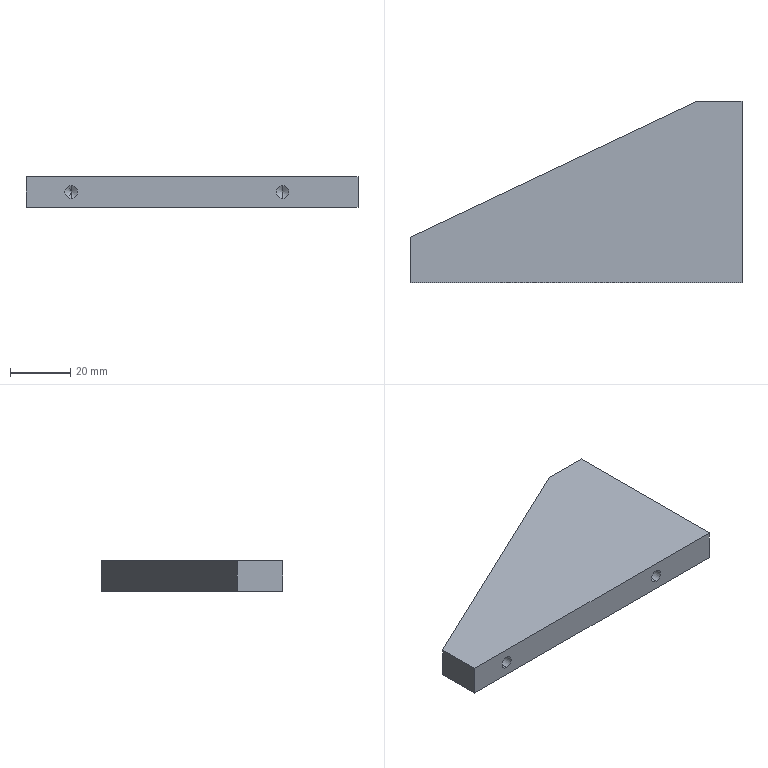Component | SolidWorks | SL021-102-4067.SL4PRT-1 | 1 solid | 23 faces | box 110 x 60 x 10 mm | volume 43715 mm3 | cylinder 8 | cone 8 | plane 7 | commonest cylinder face diameters 4.2 x8 | material AL6061
build123d program:
from build123d import *

# Parameters (mm, degrees)
BOSS_EXTRUDE1_DEPTH   = 5
M5_TAPPED_HOLE1_D     = 4.2
M5_TAPPED_HOLE1_DEPTH = 16
M5_TAPPED_HOLE1_TIP   = 1.262
M5_TAPPED_HOLE2_D     = 4.2
M5_TAPPED_HOLE2_DEPTH = 16
M5_TAPPED_HOLE2_TIP   = 1.262


with BuildPart() as part:
    # Sketch1 → Boss-Extrude1 (new, symmetric)
    with BuildSketch(Plane.XY):
        Polygon((0, 0), (0, 60), (15, 60), (110, 15), (110, 0), align=None)
    extrude(amount=BOSS_EXTRUDE1_DEPTH, both=True)

    # M5 Tapped Hole1
    with Locations(Plane.ZY):
        with Locations((0, 50), (0, 15)):
            Hole(M5_TAPPED_HOLE1_D / 2, depth=M5_TAPPED_HOLE1_DEPTH)
            with Locations((0, 0, -(M5_TAPPED_HOLE1_DEPTH + M5_TAPPED_HOLE1_TIP / 2))):  # 118° drill point
                Cone(0, M5_TAPPED_HOLE1_D / 2, M5_TAPPED_HOLE1_TIP, mode=Mode.SUBTRACT)

    # M5 Tapped Hole2
    with Locations(Plane(origin=(0, 0, 0), x_dir=(-1, 0, 0), z_dir=(0, -1, 0))):
        with Locations((-25, 0), (-95, 0)):
            Hole(M5_TAPPED_HOLE2_D / 2, depth=M5_TAPPED_HOLE2_DEPTH)
            with Locations((0, 0, -(M5_TAPPED_HOLE2_DEPTH + M5_TAPPED_HOLE2_TIP / 2))):  # 118° drill point
                Cone(0, M5_TAPPED_HOLE2_D / 2, M5_TAPPED_HOLE2_TIP, mode=Mode.SUBTRACT)


solid = part.part

# Placed as in the assembly
solid = solid.moved(Location((13.837, -10.499, -86.378), (-180, 0, 180)))
STEP:
#1=COLOUR_RGB('',0.7922,0.8196,0.9333);
#2=FILL_AREA_STYLE_COLOUR('',#1);
#3=FILL_AREA_STYLE('',(#2));
#4=SURFACE_STYLE_FILL_AREA(#3);
#5=SURFACE_SIDE_STYLE('',(#4));
#6=SURFACE_STYLE_USAGE(.BOTH.,#5);
#7=PRESENTATION_STYLE_ASSIGNMENT((#6));
#8=CARTESIAN_POINT('',(-0.4395,0.2166,-3.483));
#9=VERTEX_POINT('',#8);
#10=CARTESIAN_POINT('',(-0.4395,0.2166,-3.318));
#11=VERTEX_POINT('',#10);
#12=CARTESIAN_POINT('',(-0.4395,0.2166,-3.401));
#13=DIRECTION('',(-0.,-1.,0.));
#14=DIRECTION('',(0.,0.,1.));
#15=AXIS2_PLACEMENT_3D('',#12,#13,#14);
#16=CIRCLE('',#15,0.08268);
#17=EDGE_CURVE('',#9,#11,#16,.T.);
#18=ORIENTED_EDGE('',*,*,#17,.F.);
#19=CARTESIAN_POINT('',(-0.4395,-0.4133,-3.483));
#20=VERTEX_POINT('',#19);
#21=CARTESIAN_POINT('',(-0.4395,-0.4133,-3.483));
#22=DIRECTION('',(-0.,-1.,0.));
#23=VECTOR('',#22,39.37);
#24=LINE('',#21,#23);
#25=EDGE_CURVE('',#9,#20,#24,.T.);
#26=ORIENTED_EDGE('',*,*,#25,.T.);
#27=CARTESIAN_POINT('',(-0.4395,-0.4133,-3.318));
#28=VERTEX_POINT('',#27);
#29=CARTESIAN_POINT('',(-0.4395,-0.4133,-3.401));
#30=DIRECTION('',(-0.,-1.,0.));
#31=DIRECTION('',(0.,0.,1.));
#32=AXIS2_PLACEMENT_3D('',#29,#30,#31);
#33=CIRCLE('',#32,0.08268);
#34=EDGE_CURVE('',#20,#28,#33,.T.);
#35=ORIENTED_EDGE('',*,*,#34,.T.);
#36=CARTESIAN_POINT('',(-0.4395,-0.4133,-3.318));
#37=DIRECTION('',(-0.,-1.,0.));
#38=VECTOR('',#37,39.37);
#39=LINE('',#36,#38);
#40=EDGE_CURVE('',#11,#28,#39,.T.);
#41=ORIENTED_EDGE('',*,*,#40,.F.);
#42=EDGE_LOOP('',(#18,#26,#35,#41));
#43=FACE_OUTER_BOUND('',#42,.T.);
#44=CARTESIAN_POINT('',(-0.4395,-0.4133,-3.401));
#45=DIRECTION('',(-0.,-1.,0.));
#46=DIRECTION('',(0.,0.,1.));
#47=AXIS2_PLACEMENT_3D('',#44,#45,#46);
#48=CYLINDRICAL_SURFACE('',#47,0.08268);
#49=ADVANCED_FACE('',(#43),#48,.F.);
#50=CARTESIAN_POINT('',(-0.4395,0.2663,-3.401));
#51=VERTEX_POINT('',#50);
#52=CARTESIAN_POINT('',(-0.4395,0.2166,-3.318));
#53=DIRECTION('',(0.,-0.515,0.8572));
#54=VECTOR('',#53,39.37);
#55=LINE('',#52,#54);
#56=EDGE_CURVE('',#51,#11,#55,.T.);
#57=ORIENTED_EDGE('',*,*,#56,.F.);
#58=CARTESIAN_POINT('',(-0.4395,0.2166,-3.483));
#59=DIRECTION('',(-0.,-0.515,-0.8572));
#60=VECTOR('',#59,39.37);
#61=LINE('',#58,#60);
#62=EDGE_CURVE('',#51,#9,#61,.T.);
#63=ORIENTED_EDGE('',*,*,#62,.T.);
#64=ORIENTED_EDGE('',*,*,#17,.T.);
#65=EDGE_LOOP('',(#57,#63,#64));
#66=FACE_OUTER_BOUND('',#65,.T.);
#67=CARTESIAN_POINT('',(-0.4395,0.2166,-3.401));
#68=DIRECTION('',(-0.,-1.,0.));
#69=DIRECTION('',(0.,0.,1.));
#70=AXIS2_PLACEMENT_3D('',#67,#68,#69);
#71=CONICAL_SURFACE('',#70,0.08268,1.03);
#72=ADVANCED_FACE('',(#66),#71,.F.);
#73=CARTESIAN_POINT('',(-3.195,0.2166,-3.483));
#74=VERTEX_POINT('',#73);
#75=CARTESIAN_POINT('',(-3.195,0.2166,-3.318));
#76=VERTEX_POINT('',#75);
#77=CARTESIAN_POINT('',(-3.195,0.2166,-3.401));
#78=DIRECTION('',(-0.,-1.,0.));
#79=DIRECTION('',(0.,0.,1.));
#80=AXIS2_PLACEMENT_3D('',#77,#78,#79);
#81=CIRCLE('',#80,0.08268);
#82=EDGE_CURVE('',#74,#76,#81,.T.);
#83=ORIENTED_EDGE('',*,*,#82,.F.);
#84=CARTESIAN_POINT('',(-3.195,-0.4133,-3.483));
#85=VERTEX_POINT('',#84);
#86=CARTESIAN_POINT('',(-3.195,-0.4133,-3.483));
#87=DIRECTION('',(-0.,-1.,0.));
#88=VECTOR('',#87,39.37);
#89=LINE('',#86,#88);
#90=EDGE_CURVE('',#74,#85,#89,.T.);
#91=ORIENTED_EDGE('',*,*,#90,.T.);
#92=CARTESIAN_POINT('',(-3.195,-0.4133,-3.318));
#93=VERTEX_POINT('',#92);
#94=CARTESIAN_POINT('',(-3.195,-0.4133,-3.401));
#95=DIRECTION('',(-0.,-1.,0.));
#96=DIRECTION('',(0.,0.,1.));
#97=AXIS2_PLACEMENT_3D('',#94,#95,#96);
#98=CIRCLE('',#97,0.08268);
#99=EDGE_CURVE('',#85,#93,#98,.T.);
#100=ORIENTED_EDGE('',*,*,#99,.T.);
#101=CARTESIAN_POINT('',(-3.195,-0.4133,-3.318));
#102=DIRECTION('',(-0.,-1.,0.));
#103=VECTOR('',#102,39.37);
#104=LINE('',#101,#103);
#105=EDGE_CURVE('',#76,#93,#104,.T.);
#106=ORIENTED_EDGE('',*,*,#105,.F.);
#107=EDGE_LOOP('',(#83,#91,#100,#106));
#108=FACE_OUTER_BOUND('',#107,.T.);
#109=CARTESIAN_POINT('',(-3.195,-0.4133,-3.401));
#110=DIRECTION('',(-0.,-1.,0.));
#111=DIRECTION('',(0.,0.,1.));
#112=AXIS2_PLACEMENT_3D('',#109,#110,#111);
#113=CYLINDRICAL_SURFACE('',#112,0.08268);
#114=ADVANCED_FACE('',(#108),#113,.F.);
#115=CARTESIAN_POINT('',(-3.195,0.2663,-3.401));
#116=VERTEX_POINT('',#115);
#117=CARTESIAN_POINT('',(-3.195,0.2166,-3.318));
#118=DIRECTION('',(0.,-0.515,0.8572));
#119=VECTOR('',#118,39.37);
#120=LINE('',#117,#119);
#121=EDGE_CURVE('',#116,#76,#120,.T.);
#122=ORIENTED_EDGE('',*,*,#121,.F.);
#123=CARTESIAN_POINT('',(-3.195,0.2166,-3.483));
#124=DIRECTION('',(-0.,-0.515,-0.8572));
#125=VECTOR('',#124,39.37);
#126=LINE('',#123,#125);
#127=EDGE_CURVE('',#116,#74,#126,.T.);
#128=ORIENTED_EDGE('',*,*,#127,.T.);
#129=ORIENTED_EDGE('',*,*,#82,.T.);
#130=EDGE_LOOP('',(#122,#128,#129));
#131=FACE_OUTER_BOUND('',#130,.T.);
#132=CARTESIAN_POINT('',(-3.195,0.2166,-3.401));
#133=DIRECTION('',(-0.,-1.,0.));
#134=DIRECTION('',(0.,0.,1.));
#135=AXIS2_PLACEMENT_3D('',#132,#133,#134);
#136=CONICAL_SURFACE('',#135,0.08268,1.03);
#137=ADVANCED_FACE('',(#131),#136,.F.);
#138=CARTESIAN_POINT('',(-0.08518,1.555,-3.318));
#139=VERTEX_POINT('',#138);
#140=CARTESIAN_POINT('',(-0.08518,1.555,-3.483));
#141=VERTEX_POINT('',#140);
#142=CARTESIAN_POINT('',(-0.08518,1.555,-3.401));
#143=DIRECTION('',(1.,-0.,0.));
#144=DIRECTION('',(-0.,0.,-1.));
#145=AXIS2_PLACEMENT_3D('',#142,#143,#144);
#146=CIRCLE('',#145,0.08268);
#147=EDGE_CURVE('',#139,#141,#146,.T.);
#148=ORIENTED_EDGE('',*,*,#147,.F.);
#149=CARTESIAN_POINT('',(0.5447,1.555,-3.318));
#150=VERTEX_POINT('',#149);
#151=CARTESIAN_POINT('',(0.5447,1.555,-3.318));
#152=DIRECTION('',(1.,-0.,0.));
#153=VECTOR('',#152,39.37);
#154=LINE('',#151,#153);
#155=EDGE_CURVE('',#139,#150,#154,.T.);
#156=ORIENTED_EDGE('',*,*,#155,.T.);
#157=CARTESIAN_POINT('',(0.5447,1.555,-3.483));
#158=VERTEX_POINT('',#157);
#159=CARTESIAN_POINT('',(0.5447,1.555,-3.401));
#160=DIRECTION('',(1.,-0.,0.));
#161=DIRECTION('',(0.,0.,-1.));
#162=AXIS2_PLACEMENT_3D('',#159,#160,#161);
#163=CIRCLE('',#162,0.08268);
#164=EDGE_CURVE('',#150,#158,#163,.T.);
#165=ORIENTED_EDGE('',*,*,#164,.T.);
#166=CARTESIAN_POINT('',(0.5447,1.555,-3.483));
#167=DIRECTION('',(1.,-0.,0.));
#168=VECTOR('',#167,39.37);
#169=LINE('',#166,#168);
#170=EDGE_CURVE('',#141,#158,#169,.T.);
#171=ORIENTED_EDGE('',*,*,#170,.F.);
#172=EDGE_LOOP('',(#148,#156,#165,#171));
#173=FACE_OUTER_BOUND('',#172,.T.);
#174=CARTESIAN_POINT('',(0.5447,1.555,-3.401));
#175=DIRECTION('',(1.,-0.,0.));
#176=DIRECTION('',(0.,0.,-1.));
#177=AXIS2_PLACEMENT_3D('',#174,#175,#176);
#178=CYLINDRICAL_SURFACE('',#177,0.08268);
#179=ADVANCED_FACE('',(#173),#178,.F.);
#180=CARTESIAN_POINT('',(-0.1349,1.555,-3.401));
#181=VERTEX_POINT('',#180);
#182=CARTESIAN_POINT('',(-0.08518,1.555,-3.483));
#183=DIRECTION('',(0.515,-0.,-0.8572));
#184=VECTOR('',#183,39.37);
#185=LINE('',#182,#184);
#186=EDGE_CURVE('',#181,#141,#185,.T.);
#187=ORIENTED_EDGE('',*,*,#186,.F.);
#188=CARTESIAN_POINT('',(-0.08518,1.555,-3.318));
#189=DIRECTION('',(0.515,0.,0.8572));
#190=VECTOR('',#189,39.37);
#191=LINE('',#188,#190);
#192=EDGE_CURVE('',#181,#139,#191,.T.);
#193=ORIENTED_EDGE('',*,*,#192,.T.);
#194=ORIENTED_EDGE('',*,*,#147,.T.);
#195=EDGE_LOOP('',(#187,#193,#194));
#196=FACE_OUTER_BOUND('',#195,.T.);
#197=CARTESIAN_POINT('',(-0.08518,1.555,-3.401));
#198=DIRECTION('',(1.,-0.,0.));
#199=DIRECTION('',(-0.,0.,-1.));
#200=AXIS2_PLACEMENT_3D('',#197,#198,#199);
#201=CONICAL_SURFACE('',#200,0.08268,1.03);
#202=ADVANCED_FACE('',(#196),#201,.F.);
#203=CARTESIAN_POINT('',(-0.08518,0.1772,-3.318));
#204=VERTEX_POINT('',#203);
#205=CARTESIAN_POINT('',(-0.08518,0.1772,-3.483));
#206=VERTEX_POINT('',#205);
#207=CARTESIAN_POINT('',(-0.08518,0.1772,-3.401));
#208=DIRECTION('',(1.,-0.,0.));
#209=DIRECTION('',(-0.,0.,-1.));
#210=AXIS2_PLACEMENT_3D('',#207,#208,#209);
#211=CIRCLE('',#210,0.08268);
#212=EDGE_CURVE('',#204,#206,#211,.T.);
#213=ORIENTED_EDGE('',*,*,#212,.F.);
#214=CARTESIAN_POINT('',(0.5447,0.1772,-3.318));
#215=VERTEX_POINT('',#214);
#216=CARTESIAN_POINT('',(0.5447,0.1772,-3.318));
#217=DIRECTION('',(1.,-0.,0.));
#218=VECTOR('',#217,39.37);
#219=LINE('',#216,#218);
#220=EDGE_CURVE('',#204,#215,#219,.T.);
#221=ORIENTED_EDGE('',*,*,#220,.T.);
#222=CARTESIAN_POINT('',(0.5447,0.1772,-3.483));
#223=VERTEX_POINT('',#222);
#224=CARTESIAN_POINT('',(0.5447,0.1772,-3.401));
#225=DIRECTION('',(1.,-0.,0.));
#226=DIRECTION('',(0.,0.,-1.));
#227=AXIS2_PLACEMENT_3D('',#224,#225,#226);
#228=CIRCLE('',#227,0.08268);
#229=EDGE_CURVE('',#215,#223,#228,.T.);
#230=ORIENTED_EDGE('',*,*,#229,.T.);
#231=CARTESIAN_POINT('',(0.5447,0.1772,-3.483));
#232=DIRECTION('',(1.,-0.,0.));
#233=VECTOR('',#232,39.37);
#234=LINE('',#231,#233);
#235=EDGE_CURVE('',#206,#223,#234,.T.);
#236=ORIENTED_EDGE('',*,*,#235,.F.);
#237=EDGE_LOOP('',(#213,#221,#230,#236));
#238=FACE_OUTER_BOUND('',#237,.T.);
#239=CARTESIAN_POINT('',(0.5447,0.1772,-3.401));
#240=DIRECTION('',(1.,-0.,0.));
#241=DIRECTION('',(0.,0.,-1.));
#242=AXIS2_PLACEMENT_3D('',#239,#240,#241);
#243=CYLINDRICAL_SURFACE('',#242,0.08268);
#244=ADVANCED_FACE('',(#238),#243,.F.);
#245=CARTESIAN_POINT('',(-0.1349,0.1772,-3.401));
#246=VERTEX_POINT('',#245);
#247=CARTESIAN_POINT('',(-0.08518,0.1772,-3.483));
#248=DIRECTION('',(0.515,-0.,-0.8572));
#249=VECTOR('',#248,39.37);
#250=LINE('',#247,#249);
#251=EDGE_CURVE('',#246,#206,#250,.T.);
#252=ORIENTED_EDGE('',*,*,#251,.F.);
#253=CARTESIAN_POINT('',(-0.08518,0.1772,-3.318));
#254=DIRECTION('',(0.515,0.,0.8572));
#255=VECTOR('',#254,39.37);
#256=LINE('',#253,#255);
#257=EDGE_CURVE('',#246,#204,#256,.T.);
#258=ORIENTED_EDGE('',*,*,#257,.T.);
#259=ORIENTED_EDGE('',*,*,#212,.T.);
#260=EDGE_LOOP('',(#252,#258,#259));
#261=FACE_OUTER_BOUND('',#260,.T.);
#262=CARTESIAN_POINT('',(-0.08518,0.1772,-3.401));
#263=DIRECTION('',(1.,-0.,0.));
#264=DIRECTION('',(-0.,0.,-1.));
#265=AXIS2_PLACEMENT_3D('',#262,#263,#264);
#266=CONICAL_SURFACE('',#265,0.08268,1.03);
#267=ADVANCED_FACE('',(#261),#266,.F.);
#268=CARTESIAN_POINT('',(-0.4395,-0.4133,-3.401));
#269=DIRECTION('',(-0.,-1.,0.));
#270=DIRECTION('',(0.,0.,1.));
#271=AXIS2_PLACEMENT_3D('',#268,#269,#270);
#272=CIRCLE('',#271,0.08268);
#273=EDGE_CURVE('',#28,#20,#272,.T.);
#274=ORIENTED_EDGE('',*,*,#273,.F.);
#275=ORIENTED_EDGE('',*,*,#34,.F.);
#276=EDGE_LOOP('',(#274,#275));
#277=FACE_BOUND('',#276,.T.);
#278=CARTESIAN_POINT('',(-3.195,-0.4133,-3.401));
#279=DIRECTION('',(-0.,-1.,0.));
#280=DIRECTION('',(0.,0.,1.));
#281=AXIS2_PLACEMENT_3D('',#278,#279,#280);
#282=CIRCLE('',#281,0.08268);
#283=EDGE_CURVE('',#93,#85,#282,.T.);
#284=ORIENTED_EDGE('',*,*,#283,.F.);
#285=ORIENTED_EDGE('',*,*,#99,.F.);
#286=EDGE_LOOP('',(#284,#285));
#287=FACE_BOUND('',#286,.T.);
#288=CARTESIAN_POINT('',(0.5447,-0.4133,-3.204));
#289=VERTEX_POINT('',#288);
#290=CARTESIAN_POINT('',(-3.786,-0.4133,-3.204));
#291=VERTEX_POINT('',#290);
#292=CARTESIAN_POINT('',(-3.786,-0.4133,-3.204));
#293=DIRECTION('',(-1.,0.,-0.));
#294=VECTOR('',#293,39.37);
#295=LINE('',#292,#294);
#296=EDGE_CURVE('',#289,#291,#295,.T.);
#297=ORIENTED_EDGE('',*,*,#296,.T.);
#298=CARTESIAN_POINT('',(-3.786,-0.4133,-3.598));
#299=VERTEX_POINT('',#298);
#300=CARTESIAN_POINT('',(-3.786,-0.4133,-3.598));
#301=DIRECTION('',(0.,0.,1.));
#302=VECTOR('',#301,39.37);
#303=LINE('',#300,#302);
#304=EDGE_CURVE('',#299,#291,#303,.T.);
#305=ORIENTED_EDGE('',*,*,#304,.F.);
#306=CARTESIAN_POINT('',(0.5447,-0.4133,-3.598));
#307=VERTEX_POINT('',#306);
#308=CARTESIAN_POINT('',(-3.786,-0.4133,-3.598));
#309=DIRECTION('',(-1.,0.,-0.));
#310=VECTOR('',#309,39.37);
#311=LINE('',#308,#310);
#312=EDGE_CURVE('',#307,#299,#311,.T.);
#313=ORIENTED_EDGE('',*,*,#312,.F.);
#314=CARTESIAN_POINT('',(0.5447,-0.4133,-3.598));
#315=DIRECTION('',(0.,0.,1.));
#316=VECTOR('',#315,39.37);
#317=LINE('',#314,#316);
#318=EDGE_CURVE('',#307,#289,#317,.T.);
#319=ORIENTED_EDGE('',*,*,#318,.T.);
#320=EDGE_LOOP('',(#297,#305,#313,#319));
#321=FACE_OUTER_BOUND('',#320,.T.);
#322=CARTESIAN_POINT('',(-3.786,-0.4133,-3.598));
#323=DIRECTION('',(0.,1.,-0.));
#324=DIRECTION('',(1.,-0.,0.));
#325=AXIS2_PLACEMENT_3D('',#322,#323,#324);
#326=PLANE('',#325);
#327=ADVANCED_FACE('',(#277,#287,#321),#326,.F.);
#328=CARTESIAN_POINT('',(-3.786,0.1772,-3.204));
#329=VERTEX_POINT('',#328);
#330=CARTESIAN_POINT('',(-3.786,0.1772,-3.204));
#331=DIRECTION('',(0.,1.,-0.));
#332=VECTOR('',#331,39.37);
#333=LINE('',#330,#332);
#334=EDGE_CURVE('',#291,#329,#333,.T.);
#335=ORIENTED_EDGE('',*,*,#334,.T.);
#336=CARTESIAN_POINT('',(-3.786,0.1772,-3.598));
#337=VERTEX_POINT('',#336);
#338=CARTESIAN_POINT('',(-3.786,0.1772,-3.598));
#339=DIRECTION('',(0.,0.,1.));
#340=VECTOR('',#339,39.37);
#341=LINE('',#338,#340);
#342=EDGE_CURVE('',#337,#329,#341,.T.);
#343=ORIENTED_EDGE('',*,*,#342,.F.);
#344=CARTESIAN_POINT('',(-3.786,0.1772,-3.598));
#345=DIRECTION('',(0.,1.,-0.));
#346=VECTOR('',#345,39.37);
#347=LINE('',#344,#346);
#348=EDGE_CURVE('',#299,#337,#347,.T.);
#349=ORIENTED_EDGE('',*,*,#348,.F.);
#350=ORIENTED_EDGE('',*,*,#304,.T.);
#351=EDGE_LOOP('',(#335,#343,#349,#350));
#352=FACE_OUTER_BOUND('',#351,.T.);
#353=CARTESIAN_POINT('',(-3.786,0.1772,-3.598));
#354=DIRECTION('',(1.,-0.,-0.));
#355=DIRECTION('',(-0.,-0.,-1.));
#356=AXIS2_PLACEMENT_3D('',#353,#354,#355);
#357=PLANE('',#356);
#358=ADVANCED_FACE('',(#352),#357,.F.);
#359=CARTESIAN_POINT('',(-0.04581,1.949,-3.204));
#360=VERTEX_POINT('',#359);
#361=CARTESIAN_POINT('',(-0.04581,1.949,-3.204));
#362=DIRECTION('',(0.9037,0.4281,0.));
#363=VECTOR('',#362,39.37);
#364=LINE('',#361,#363);
#365=EDGE_CURVE('',#329,#360,#364,.T.);
#366=ORIENTED_EDGE('',*,*,#365,.T.);
#367=CARTESIAN_POINT('',(-0.04581,1.949,-3.598));
#368=VERTEX_POINT('',#367);
#369=CARTESIAN_POINT('',(-0.04581,1.949,-3.598));
#370=DIRECTION('',(0.,0.,1.));
#371=VECTOR('',#370,39.37);
#372=LINE('',#369,#371);
#373=EDGE_CURVE('',#368,#360,#372,.T.);
#374=ORIENTED_EDGE('',*,*,#373,.F.);
#375=CARTESIAN_POINT('',(-0.04581,1.949,-3.598));
#376=DIRECTION('',(0.9037,0.4281,0.));
#377=VECTOR('',#376,39.37);
#378=LINE('',#375,#377);
#379=EDGE_CURVE('',#337,#368,#378,.T.);
#380=ORIENTED_EDGE('',*,*,#379,.F.);
#381=ORIENTED_EDGE('',*,*,#342,.T.);
#382=EDGE_LOOP('',(#366,#374,#380,#381));
#383=FACE_OUTER_BOUND('',#382,.T.);
#384=CARTESIAN_POINT('',(-0.04581,1.949,-3.598));
#385=DIRECTION('',(0.4281,-0.9037,0.));
#386=DIRECTION('',(-0.9037,-0.4281,-0.));
#387=AXIS2_PLACEMENT_3D('',#384,#385,#386);
#388=PLANE('',#387);
#389=ADVANCED_FACE('',(#383),#388,.F.);
#390=CARTESIAN_POINT('',(0.5447,1.949,-3.204));
#391=VERTEX_POINT('',#390);
#392=CARTESIAN_POINT('',(0.5447,1.949,-3.204));
#393=DIRECTION('',(1.,-0.,0.));
#394=VECTOR('',#393,39.37);
#395=LINE('',#392,#394);
#396=EDGE_CURVE('',#360,#391,#395,.T.);
#397=ORIENTED_EDGE('',*,*,#396,.T.);
#398=CARTESIAN_POINT('',(0.5447,1.949,-3.598));
#399=VERTEX_POINT('',#398);
#400=CARTESIAN_POINT('',(0.5447,1.949,-3.598));
#401=DIRECTION('',(0.,0.,1.));
#402=VECTOR('',#401,39.37);
#403=LINE('',#400,#402);
#404=EDGE_CURVE('',#399,#391,#403,.T.);
#405=ORIENTED_EDGE('',*,*,#404,.F.);
#406=CARTESIAN_POINT('',(0.5447,1.949,-3.598));
#407=DIRECTION('',(1.,-0.,0.));
#408=VECTOR('',#407,39.37);
#409=LINE('',#406,#408);
#410=EDGE_CURVE('',#368,#399,#409,.T.);
#411=ORIENTED_EDGE('',*,*,#410,.F.);
#412=ORIENTED_EDGE('',*,*,#373,.T.);
#413=EDGE_LOOP('',(#397,#405,#411,#412));
#414=FACE_OUTER_BOUND('',#413,.T.);
#415=CARTESIAN_POINT('',(0.5447,1.949,-3.598));
#416=DIRECTION('',(-0.,-1.,0.));
#417=DIRECTION('',(0.,0.,1.));
#418=AXIS2_PLACEMENT_3D('',#415,#416,#417);
#419=PLANE('',#418);
#420=ADVANCED_FACE('',(#414),#419,.F.);
#421=CARTESIAN_POINT('',(0.5447,1.555,-3.401));
#422=DIRECTION('',(1.,-0.,0.));
#423=DIRECTION('',(0.,0.,-1.));
#424=AXIS2_PLACEMENT_3D('',#421,#422,#423);
#425=CIRCLE('',#424,0.08268);
#426=EDGE_CURVE('',#158,#150,#425,.T.);
#427=ORIENTED_EDGE('',*,*,#426,.F.);
#428=ORIENTED_EDGE('',*,*,#164,.F.);
#429=EDGE_LOOP('',(#427,#428));
#430=FACE_BOUND('',#429,.T.);
#431=CARTESIAN_POINT('',(0.5447,0.1772,-3.401));
#432=DIRECTION('',(1.,-0.,0.));
#433=DIRECTION('',(0.,0.,-1.));
#434=AXIS2_PLACEMENT_3D('',#431,#432,#433);
#435=CIRCLE('',#434,0.08268);
#436=EDGE_CURVE('',#223,#215,#435,.T.);
#437=ORIENTED_EDGE('',*,*,#436,.F.);
#438=ORIENTED_EDGE('',*,*,#229,.F.);
#439=EDGE_LOOP('',(#437,#438));
#440=FACE_BOUND('',#439,.T.);
#441=CARTESIAN_POINT('',(0.5447,-0.4133,-3.204));
#442=DIRECTION('',(-0.,-1.,0.));
#443=VECTOR('',#442,39.37);
#444=LINE('',#441,#443);
#445=EDGE_CURVE('',#391,#289,#444,.T.);
#446=ORIENTED_EDGE('',*,*,#445,.T.);
#447=ORIENTED_EDGE('',*,*,#318,.F.);
#448=CARTESIAN_POINT('',(0.5447,-0.4133,-3.598));
#449=DIRECTION('',(-0.,-1.,0.));
#450=VECTOR('',#449,39.37);
#451=LINE('',#448,#450);
#452=EDGE_CURVE('',#399,#307,#451,.T.);
#453=ORIENTED_EDGE('',*,*,#452,.F.);
#454=ORIENTED_EDGE('',*,*,#404,.T.);
#455=EDGE_LOOP('',(#446,#447,#453,#454));
#456=FACE_OUTER_BOUND('',#455,.T.);
#457=CARTESIAN_POINT('',(0.5447,-0.4133,-3.598));
#458=DIRECTION('',(-1.,0.,0.));
#459=DIRECTION('',(0.,0.,1.));
#460=AXIS2_PLACEMENT_3D('',#457,#458,#459);
#461=PLANE('',#460);
#462=ADVANCED_FACE('',(#430,#440,#456),#461,.F.);
#463=ORIENTED_EDGE('',*,*,#312,.T.);
#464=ORIENTED_EDGE('',*,*,#348,.T.);
#465=ORIENTED_EDGE('',*,*,#379,.T.);
#466=ORIENTED_EDGE('',*,*,#410,.T.);
#467=ORIENTED_EDGE('',*,*,#452,.T.);
#468=EDGE_LOOP('',(#463,#464,#465,#466,#467));
#469=FACE_OUTER_BOUND('',#468,.T.);
#470=CARTESIAN_POINT('',(0.5447,-0.4133,-3.598));
#471=DIRECTION('',(-0.,0.,1.));
#472=DIRECTION('',(1.,-0.,0.));
#473=AXIS2_PLACEMENT_3D('',#470,#471,#472);
#474=PLANE('',#473);
#475=ADVANCED_FACE('',(#469),#474,.F.);
#476=ORIENTED_EDGE('',*,*,#296,.F.);
#477=ORIENTED_EDGE('',*,*,#445,.F.);
#478=ORIENTED_EDGE('',*,*,#396,.F.);
#479=ORIENTED_EDGE('',*,*,#365,.F.);
#480=ORIENTED_EDGE('',*,*,#334,.F.);
#481=EDGE_LOOP('',(#476,#477,#478,#479,#480));
#482=FACE_OUTER_BOUND('',#481,.T.);
#483=CARTESIAN_POINT('',(0.5447,-0.4133,-3.204));
#484=DIRECTION('',(-0.,0.,1.));
#485=DIRECTION('',(1.,-0.,0.));
#486=AXIS2_PLACEMENT_3D('',#483,#484,#485);
#487=PLANE('',#486);
#488=ADVANCED_FACE('',(#482),#487,.T.);
#489=ORIENTED_EDGE('',*,*,#257,.F.);
#490=ORIENTED_EDGE('',*,*,#251,.T.);
#491=CARTESIAN_POINT('',(-0.08518,0.1772,-3.401));
#492=DIRECTION('',(1.,-0.,0.));
#493=DIRECTION('',(-0.,0.,-1.));
#494=AXIS2_PLACEMENT_3D('',#491,#492,#493);
#495=CIRCLE('',#494,0.08268);
#496=EDGE_CURVE('',#206,#204,#495,.T.);
#497=ORIENTED_EDGE('',*,*,#496,.T.);
#498=EDGE_LOOP('',(#489,#490,#497));
#499=FACE_OUTER_BOUND('',#498,.T.);
#500=CARTESIAN_POINT('',(-0.08518,0.1772,-3.401));
#501=DIRECTION('',(1.,-0.,0.));
#502=DIRECTION('',(-0.,0.,-1.));
#503=AXIS2_PLACEMENT_3D('',#500,#501,#502);
#504=CONICAL_SURFACE('',#503,0.08268,1.03);
#505=ADVANCED_FACE('',(#499),#504,.F.);
#506=ORIENTED_EDGE('',*,*,#220,.F.);
#507=ORIENTED_EDGE('',*,*,#496,.F.);
#508=ORIENTED_EDGE('',*,*,#235,.T.);
#509=ORIENTED_EDGE('',*,*,#436,.T.);
#510=EDGE_LOOP('',(#506,#507,#508,#509));
#511=FACE_OUTER_BOUND('',#510,.T.);
#512=CARTESIAN_POINT('',(0.5447,0.1772,-3.401));
#513=DIRECTION('',(1.,-0.,0.));
#514=DIRECTION('',(0.,0.,-1.));
#515=AXIS2_PLACEMENT_3D('',#512,#513,#514);
#516=CYLINDRICAL_SURFACE('',#515,0.08268);
#517=ADVANCED_FACE('',(#511),#516,.F.);
#518=ORIENTED_EDGE('',*,*,#192,.F.);
#519=ORIENTED_EDGE('',*,*,#186,.T.);
#520=CARTESIAN_POINT('',(-0.08518,1.555,-3.401));
#521=DIRECTION('',(1.,-0.,0.));
#522=DIRECTION('',(-0.,0.,-1.));
#523=AXIS2_PLACEMENT_3D('',#520,#521,#522);
#524=CIRCLE('',#523,0.08268);
#525=EDGE_CURVE('',#141,#139,#524,.T.);
#526=ORIENTED_EDGE('',*,*,#525,.T.);
#527=EDGE_LOOP('',(#518,#519,#526));
#528=FACE_OUTER_BOUND('',#527,.T.);
#529=CARTESIAN_POINT('',(-0.08518,1.555,-3.401));
#530=DIRECTION('',(1.,-0.,0.));
#531=DIRECTION('',(-0.,0.,-1.));
#532=AXIS2_PLACEMENT_3D('',#529,#530,#531);
#533=CONICAL_SURFACE('',#532,0.08268,1.03);
#534=ADVANCED_FACE('',(#528),#533,.F.);
#535=ORIENTED_EDGE('',*,*,#155,.F.);
#536=ORIENTED_EDGE('',*,*,#525,.F.);
#537=ORIENTED_EDGE('',*,*,#170,.T.);
#538=ORIENTED_EDGE('',*,*,#426,.T.);
#539=EDGE_LOOP('',(#535,#536,#537,#538));
#540=FACE_OUTER_BOUND('',#539,.T.);
#541=CARTESIAN_POINT('',(0.5447,1.555,-3.401));
#542=DIRECTION('',(1.,-0.,0.));
#543=DIRECTION('',(0.,0.,-1.));
#544=AXIS2_PLACEMENT_3D('',#541,#542,#543);
#545=CYLINDRICAL_SURFACE('',#544,0.08268);
#546=ADVANCED_FACE('',(#540),#545,.F.);
#547=ORIENTED_EDGE('',*,*,#127,.F.);
#548=ORIENTED_EDGE('',*,*,#121,.T.);
#549=CARTESIAN_POINT('',(-3.195,0.2166,-3.401));
#550=DIRECTION('',(-0.,-1.,0.));
#551=DIRECTION('',(0.,0.,1.));
#552=AXIS2_PLACEMENT_3D('',#549,#550,#551);
#553=CIRCLE('',#552,0.08268);
#554=EDGE_CURVE('',#76,#74,#553,.T.);
#555=ORIENTED_EDGE('',*,*,#554,.T.);
#556=EDGE_LOOP('',(#547,#548,#555));
#557=FACE_OUTER_BOUND('',#556,.T.);
#558=CARTESIAN_POINT('',(-3.195,0.2166,-3.401));
#559=DIRECTION('',(-0.,-1.,0.));
#560=DIRECTION('',(0.,0.,1.));
#561=AXIS2_PLACEMENT_3D('',#558,#559,#560);
#562=CONICAL_SURFACE('',#561,0.08268,1.03);
#563=ADVANCED_FACE('',(#557),#562,.F.);
#564=ORIENTED_EDGE('',*,*,#90,.F.);
#565=ORIENTED_EDGE('',*,*,#554,.F.);
#566=ORIENTED_EDGE('',*,*,#105,.T.);
#567=ORIENTED_EDGE('',*,*,#283,.T.);
#568=EDGE_LOOP('',(#564,#565,#566,#567));
#569=FACE_OUTER_BOUND('',#568,.T.);
#570=CARTESIAN_POINT('',(-3.195,-0.4133,-3.401));
#571=DIRECTION('',(-0.,-1.,0.));
#572=DIRECTION('',(0.,0.,1.));
#573=AXIS2_PLACEMENT_3D('',#570,#571,#572);
#574=CYLINDRICAL_SURFACE('',#573,0.08268);
#575=ADVANCED_FACE('',(#569),#574,.F.);
#576=ORIENTED_EDGE('',*,*,#62,.F.);
#577=ORIENTED_EDGE('',*,*,#56,.T.);
#578=CARTESIAN_POINT('',(-0.4395,0.2166,-3.401));
#579=DIRECTION('',(-0.,-1.,0.));
#580=DIRECTION('',(0.,0.,1.));
#581=AXIS2_PLACEMENT_3D('',#578,#579,#580);
#582=CIRCLE('',#581,0.08268);
#583=EDGE_CURVE('',#11,#9,#582,.T.);
#584=ORIENTED_EDGE('',*,*,#583,.T.);
#585=EDGE_LOOP('',(#576,#577,#584));
#586=FACE_OUTER_BOUND('',#585,.T.);
#587=CARTESIAN_POINT('',(-0.4395,0.2166,-3.401));
#588=DIRECTION('',(-0.,-1.,0.));
#589=DIRECTION('',(0.,0.,1.));
#590=AXIS2_PLACEMENT_3D('',#587,#588,#589);
#591=CONICAL_SURFACE('',#590,0.08268,1.03);
#592=ADVANCED_FACE('',(#586),#591,.F.);
#593=ORIENTED_EDGE('',*,*,#25,.F.);
#594=ORIENTED_EDGE('',*,*,#583,.F.);
#595=ORIENTED_EDGE('',*,*,#40,.T.);
#596=ORIENTED_EDGE('',*,*,#273,.T.);
#597=EDGE_LOOP('',(#593,#594,#595,#596));
#598=FACE_OUTER_BOUND('',#597,.T.);
#599=CARTESIAN_POINT('',(-0.4395,-0.4133,-3.401));
#600=DIRECTION('',(-0.,-1.,0.));
#601=DIRECTION('',(0.,0.,1.));
#602=AXIS2_PLACEMENT_3D('',#599,#600,#601);
#603=CYLINDRICAL_SURFACE('',#602,0.08268);
#604=ADVANCED_FACE('',(#598),#603,.F.);
#605=CLOSED_SHELL('',(#49,#72,#114,#137,#179,#202,#244,#267,#327,#358,#389,#420,#462,#475,#488,#505,#517,#534,#546,#563,#575,#592,#604));
#606=MANIFOLD_SOLID_BREP('',#605);
#607=STYLED_ITEM('',(#7),#606);
#608=PRESENTATION_LAYER_ASSIGNMENT('','',(#607));
#609=(LENGTH_UNIT()NAMED_UNIT(*)SI_UNIT($,.METRE.));
#610=LENGTH_MEASURE_WITH_UNIT(LENGTH_MEASURE(0.0254),#609);
#611=DIMENSIONAL_EXPONENTS(1.,0.,0.,0.,0.,0.,0.);
#612=(CONVERSION_BASED_UNIT('',#610)LENGTH_UNIT()NAMED_UNIT(#611));
#613=UNCERTAINTY_MEASURE_WITH_UNIT(LENGTH_MEASURE(0.00001),#612,'','');
#614=(NAMED_UNIT(*)PLANE_ANGLE_UNIT()SI_UNIT($,.RADIAN.));
#615=(NAMED_UNIT(*)SI_UNIT($,.STERADIAN.)SOLID_ANGLE_UNIT());
#616=(GEOMETRIC_REPRESENTATION_CONTEXT(3)GLOBAL_UNCERTAINTY_ASSIGNED_CONTEXT((#613))GLOBAL_UNIT_ASSIGNED_CONTEXT((#612,#614,#615))REPRESENTATION_CONTEXT('',''));
#617=MECHANICAL_DESIGN_GEOMETRIC_PRESENTATION_REPRESENTATION('',(#607),#616);
#618=CARTESIAN_POINT('',(0.,0.,0.));
#619=DIRECTION('',(0.,0.,1.));
#620=DIRECTION('',(1.,0.,0.));
#621=AXIS2_PLACEMENT_3D('',#618,#619,#620);
#622=(LENGTH_UNIT()NAMED_UNIT(*)SI_UNIT($,.METRE.));
#623=LENGTH_MEASURE_WITH_UNIT(LENGTH_MEASURE(0.0254),#622);
#624=DIMENSIONAL_EXPONENTS(1.,0.,0.,0.,0.,0.,0.);
#625=(CONVERSION_BASED_UNIT('',#623)LENGTH_UNIT()NAMED_UNIT(#624));
#626=UNCERTAINTY_MEASURE_WITH_UNIT(LENGTH_MEASURE(0.00001),#625,'','');
#627=(NAMED_UNIT(*)PLANE_ANGLE_UNIT()SI_UNIT($,.RADIAN.));
#628=(NAMED_UNIT(*)SI_UNIT($,.STERADIAN.)SOLID_ANGLE_UNIT());
#629=(GEOMETRIC_REPRESENTATION_CONTEXT(3)GLOBAL_UNCERTAINTY_ASSIGNED_CONTEXT((#626))GLOBAL_UNIT_ASSIGNED_CONTEXT((#625,#627,#628))REPRESENTATION_CONTEXT('',''));
#630=ADVANCED_BREP_SHAPE_REPRESENTATION('',(#606,#621),#629);